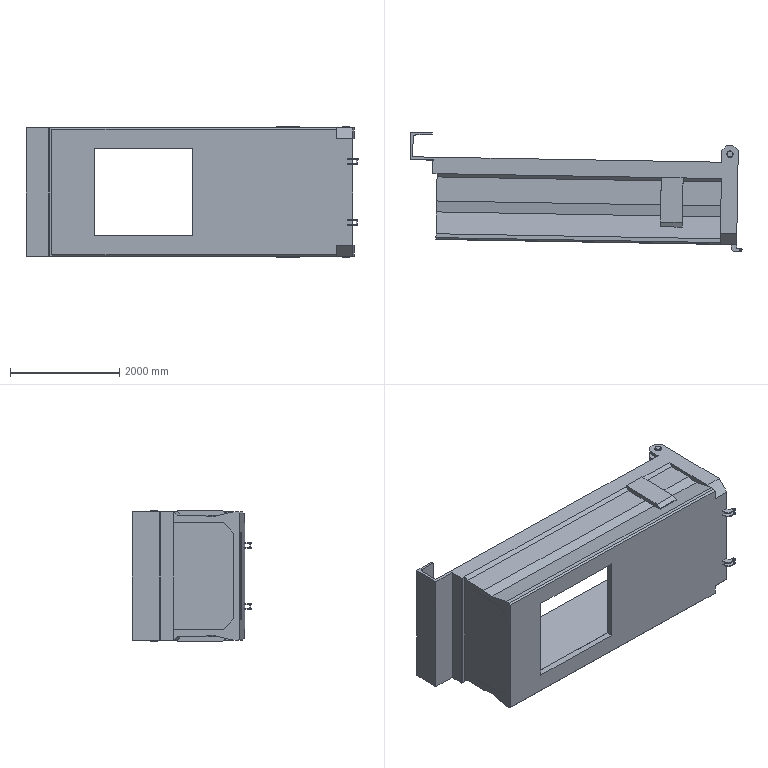Component | SolidWorks | CargoBox-1 | 3 solids | 192 faces | box 6072.17 x 2185.91 x 2410 mm | volume 3913118645 mm3 | plane 125 | cylinder 51 | cone 16 | commonest cylinder face diameters 40 x20 120 x8 30 x8 80 x6 20 x6 100 x3
build123d program:
from build123d import *

# Parameters (mm, degrees)
BOSS_EXTRUDE1_DEPTH      = 2600
SKETCH3_W                = 1950
SKETCH3_H                = 1400
BOSS_EXTRUDE2_DEPTH      = 8
SKETCH4_W                = 2350
SKETCH4_H                = 250
BOSS_EXTRUDE3_DEPTH      = 80
FILLET1_R                = 10
BOSS_EXTRUDE4_DEPTH      = 300
SKETCH6_W                = 400
SKETCH6_H                = 900
BOSS_EXTRUDE5_DEPTH      = 80
CHAMFER1_SIZE            = 50
CHAMFER1_SIZE2           = 86.603
CHAMFER2_SIZE            = 90
CHAMFER2_SIZE2           = 51.962
CUT_EXTRUDE1_DEPTH       = 390
CHAMFER3_SIZE            = 190
BOSS_EXTRUDE7_DEPTH      = 2350
FILLET2_R                = 50
CHAMFER4_SIZE            = 80
SKETCH11_W               = 80
SKETCH11_H               = 300
CUT_EXTRUDE2_DEPTH       = 390
SKETCH12_R               = 40
CUT_EXTRUDE3_DEPTH       = 4319.495
BOSS_EXTRUDE8_REACH      = 4214.054
SKETCH13_R               = 40
CHAMFER5_SIZE            = 30
BOSS_EXTRUDE9_DEPTH      = 20
SKETCH15_R               = 10
CUT_EXTRUDE4_DEPTH       = 4036.035
SKETCH16_R               = 60
BOSS_EXTRUDE10_DEPTH     = 30
BOSS_EXTRUDE12_START     = 200
SKETCH18_R               = 40
BOSS_EXTRUDE12_DEPTH     = 200
BOSS_EXTRUDE11_START     = 30
SKETCH17_R               = 60
BOSS_EXTRUDE11_DEPTH     = 30
CHAMFER6_SIZE            = 10
CHAMFER6_OF_MIRROR2_SIZE = 10
SKETCH19_R               = 15
BOSS_EXTRUDE13_DEPTH     = 10
SKETCH20_R               = 10
BOSS_EXTRUDE14_DEPTH     = 100
CHAMFER7_SIZE            = 2
CHAMFER7_OF_MIRROR9_SIZE = 2
LPATTERN1_COUNT          = 2
LPATTERN1_PITCH          = 1115
CUT_EXTRUDE5_DEPTH       = 3806.854
CUT_EXTRUDE5_DEPTH_BACK  = 3806.854
SKETCH23_W               = 1601
SKETCH23_H               = 1804


with BuildPart() as part:
    # Sketch1 → Boss-Extrude1 (new, symmetric)
    with BuildSketch(Plane.XY):
        Polygon((-975, 1400), (-975, 0), (975, 0), (975, 1400), (1175, 1400), (1175, 1100), (1115, 1040), (1115, 600), (1079.735, 400), (1175, 0), (1175, -100), (-1175, -100), (-1175, 0), (-1079.735, 400), (-1115, 600), (-1115, 1040), (-1175, 1100), (-1175, 1400), align=None)
    extrude(amount=BOSS_EXTRUDE1_DEPTH, both=True)

    # Sketch3 → Boss-Extrude2 (add)
    with BuildSketch(Plane(origin=(0, 0, -2600), x_dir=(-1, 0, 0), z_dir=(0, 0, -1))):
        with Locations((0, 700)):
            Rectangle(SKETCH3_W, SKETCH3_H)
    extrude(amount=-BOSS_EXTRUDE2_DEPTH)

    # Sketch5 → Boss-Extrude4 (add)
    with BuildSketch(Plane.XY.offset(2600)):
        Polygon((-1175, 1700), (-1175, 100), (-975, -100), (975, -100), (1175, 100), (1175, 1700), align=None)
    extrude(amount=BOSS_EXTRUDE4_DEPTH)

    # Sketch6 → Boss-Extrude5 (add)
    with BuildSketch(Plane.ZY.offset(1115)):
        with Locations((1700, 650)):
            Rectangle(SKETCH6_W, SKETCH6_H)
    boss_extrude5 = extrude(amount=BOSS_EXTRUDE5_DEPTH)

    # Mirror1: Boss-Extrude5 across plane
    add(boss_extrude5.mirror(Plane(origin=(0, 0, 0), x_dir=(0, 0, 1), z_dir=(1, 0, 0))))

    # Chamfer1
    chamfer1_edges = [part.edges().sort_by_distance(p)[0] for p in [
        (-1195, 200, 1700),
    ]]
    chamfer1_side = [part.faces().sort_by_distance(p)[0] for p in [
        (-1161.184, 200, 1700),
    ]]
    chamfer(chamfer1_edges, length=CHAMFER1_SIZE, length2=CHAMFER1_SIZE2, reference=chamfer1_side[0])

    # Chamfer2
    chamfer2_edges = [part.edges().sort_by_distance(p)[0] for p in [
        (1195, 200, 1700),
    ]]
    chamfer2_side = [part.faces().sort_by_distance(p)[0] for p in [
        (1195, 650, 1700),
    ]]
    chamfer(chamfer2_edges, length=CHAMFER2_SIZE, length2=CHAMFER2_SIZE2, reference=chamfer2_side[0])

    # Sketch7 → Cut-Extrude1 (cut)
    with BuildSketch(Plane.XY.offset(2900)):
        Polygon((-975, 1700), (-975, 182.843), (-792.157, 0), (792.157, 0), (975, 182.843), (975, 1700), align=None)
    extrude(amount=-CUT_EXTRUDE1_DEPTH, mode=Mode.SUBTRACT)

    # Chamfer3
    chamfer3_edges = [part.edges().sort_by_distance(p)[0] for p in [
        (975, 0, 4),
        (-975, 0, 4),
    ]]
    chamfer(chamfer3_edges, length=CHAMFER3_SIZE)



with BuildPart() as body_2:
    # Sketch4 → Boss-Extrude3 (new body)
    with BuildSketch(Plane(origin=(0, 0, -2600), x_dir=(-1, 0, 0), z_dir=(0, 0, -1))):
        with Locations((0, 1225)):
            Rectangle(SKETCH4_W, SKETCH4_H)
    extrude(amount=BOSS_EXTRUDE3_DEPTH)

    # Fillet1
    fillet1_edges = [body_2.edges().sort_by_distance(p)[0] for p in [
        (0, 1350, -2680),
        (0, 1100, -2680),
    ]]
    fillet(fillet1_edges, radius=FILLET1_R)


with BuildPart() as part_1:
    add(part.part)

    add(body_2.part)  # Boss-Extrude7 merges body 2
    # Sketch9 → Boss-Extrude7 (add)
    with BuildSketch(Plane(origin=(1175, 0, 0), x_dir=(0, 0, -1), z_dir=(1, 0, 0))):
        with BuildLine():
            Line((2600, 1350), (3100, 1350))
            Line((3100, 1350), (3100, 1850))
            Line((3100, 1850), (2700, 1850))
            Line((2700, 1850), (2700, 1820))
            Line((2700, 1820), (3002.617, 1804.141))
            ThreePointArc((3002.617, 1804.141), (3036.269, 1788.627), (3050, 1754.209))
            Line((3050, 1754.209), (3050, 1400))
            Line((3050, 1400), (2600, 1400))
            Line((2600, 1400), (2600, 1350))
        make_face()
    extrude(amount=-BOSS_EXTRUDE7_DEPTH)

    # Fillet2
    fillet2_edges = [part_1.edges().sort_by_distance(p)[0] for p in [
        (1175, 1835, -2700),
        (-1175, 1835, -2700),
    ]]
    fillet(fillet2_edges, radius=FILLET2_R)

    # Chamfer4
    chamfer4_edges = [part_1.edges().sort_by_distance(p)[0] for p in [
        (1075, 1700, 2600),
        (-1075, 1700, 2600),
        (1075, 1700, 2900),
        (-1075, 1700, 2900),
    ]]
    chamfer(chamfer4_edges, length=CHAMFER4_SIZE)

    # Sketch11 → Cut-Extrude2 (cut)
    with BuildSketch(Plane.XY.offset(2900)):
        with Locations((1075, 1550)):
            Rectangle(SKETCH11_W, SKETCH11_H)
        with Locations((-1075, 1550)):
            Rectangle(SKETCH11_W, SKETCH11_H)
    extrude(amount=-CUT_EXTRUDE2_DEPTH, mode=Mode.SUBTRACT)

    # Sketch12 → Cut-Extrude3 (cut, through all)
    with BuildSketch(Plane(origin=(1175, 0, 0), x_dir=(0, 0, -1), z_dir=(1, 0, 0))):
        with Locations((-2750, 1550)):
            Circle(SKETCH12_R)
    extrude(amount=-CUT_EXTRUDE3_DEPTH, mode=Mode.SUBTRACT)

    # Sketch13 → Boss-Extrude8 (add, up to next)
    with BuildSketch(Plane(origin=(-975, 0, 0), x_dir=(0, 0, -1), z_dir=(1, 0, 0)), mode=Mode.PRIVATE) as boss_extrude8_sk1:
        with Locations(Location((-2300, 1200, 0), (0, 0, 180))):
            Circle(SKETCH13_R)
    boss_extrude8_tool1 = extrude(boss_extrude8_sk1.sketch, amount=BOSS_EXTRUDE8_REACH, mode=Mode.PRIVATE) - part_1.part
    add(boss_extrude8_tool1.solids().sort_by_distance((-975, 1200, 2300))[0])

    # Chamfer5
    chamfer5_edges = [part_1.edges().sort_by_distance(p)[0] for p in [
        (-1175, -100, 0),
        (1175, -100, 0),
    ]]
    chamfer(chamfer5_edges, length=CHAMFER5_SIZE)

    # Sketch16 → Boss-Extrude10 (add)
    with BuildSketch(Plane.ZY.offset(1175)):
        with Locations(Location((2750, 1550, 0), (0, 0, 180))):
            Circle(SKETCH16_R)
    boss_extrude10 = extrude(amount=BOSS_EXTRUDE10_DEPTH)

    # Sketch18 → Boss-Extrude12 (add)
    with BuildSketch(Plane(origin=(-1175, 0, 0), x_dir=(0, 0, -1), z_dir=(1, 0, 0)).offset(BOSS_EXTRUDE12_START)):
        with Locations((-2750, 1550)):
            Circle(SKETCH18_R)
    boss_extrude12 = extrude(amount=-BOSS_EXTRUDE12_DEPTH)

    # Sketch17 → Boss-Extrude11 (add)
    with BuildSketch(Plane(origin=(-975, 0, 0), x_dir=(0, 0, -1), z_dir=(1, 0, 0)).offset(BOSS_EXTRUDE11_START)):
        with Locations((-2750, 1550)):
            Circle(SKETCH17_R)
    boss_extrude11 = extrude(amount=-BOSS_EXTRUDE11_DEPTH)

    # Chamfer6
    chamfer6_edges = [part_1.edges().sort_by_distance(p)[0] for p in [
        (-1205, 1550, 2810),
        (-945, 1550, 2810),
    ]]
    chamfer(chamfer6_edges, length=CHAMFER6_SIZE)

    # Mirror2: Boss-Extrude10, Boss-Extrude12, Boss-Extrude11 across plane
    add(boss_extrude10.mirror(Plane(origin=(0, 0, 0), x_dir=(0, 0, 1), z_dir=(1, 0, 0))))
    add(boss_extrude12.mirror(Plane(origin=(0, 0, 0), x_dir=(0, 0, 1), z_dir=(1, 0, 0))))
    add(boss_extrude11.mirror(Plane(origin=(0, 0, 0), x_dir=(0, 0, 1), z_dir=(1, 0, 0))))

    # Chamfer6 of Mirror2
    chamfer6_of_mirror2_edges = [part_1.edges().sort_by_distance(p)[0] for p in [
        (1205, 1550, 2810),
        (945, 1550, 2810),
    ]]
    chamfer(chamfer6_of_mirror2_edges, length=CHAMFER6_OF_MIRROR2_SIZE)

    # Sketch23 → Cut-Extrude5 (cut, two sides: drawn at the far end of the back side and taken through both)
    with BuildSketch(Plane(origin=(0, 0, 0), x_dir=(1, 0, 0), z_dir=(0, 1, 0)).offset(-CUT_EXTRUDE5_DEPTH_BACK)):
        with Locations((0, 926.743)):
            Rectangle(SKETCH23_W, SKETCH23_H)
    extrude(amount=CUT_EXTRUDE5_DEPTH + CUT_EXTRUDE5_DEPTH_BACK, mode=Mode.SUBTRACT)


with BuildPart() as body_2_2:
    # Sketch14 → Boss-Extrude9 (new body)
    with BuildSketch(Plane.ZY.offset(607.5)):
        with BuildLine():
            Line((2800, -100), (2900, -100))
            Line((2900, -100), (2900, -150))
            ThreePointArc((2900, -150), (2905.858, -164.142), (2920, -170))
            Line((2920, -170), (2980, -170))
            ThreePointArc((2980, -170), (2994.142, -175.858), (3000, -190))
            Line((3000, -190), (3000, -210))
            ThreePointArc((3000, -210), (2994.142, -224.142), (2980, -230))
            Line((2980, -230), (2858.284, -230))
            ThreePointArc((2858.284, -230), (2850.631, -228.478), (2844.142, -224.142))
            Line((2844.142, -224.142), (2805.858, -185.858))
            ThreePointArc((2805.858, -185.858), (2801.522, -179.369), (2800, -171.716))
            Line((2800, -171.716), (2800, -100))
        make_face()
    extrude(amount=-BOSS_EXTRUDE9_DEPTH)

    # Sketch15 → Cut-Extrude4 (cut, through all)
    with BuildSketch(Plane.ZY.offset(607.5)):
        with Locations((2975, -200)):
            Circle(SKETCH15_R)
    extrude(amount=-CUT_EXTRUDE4_DEPTH, mode=Mode.SUBTRACT)


with BuildPart() as body_3:
    # Body-Move_Copy1: copy of body 2 2
    add(body_2_2.part.moved(Location((80, 0, 0))))


with BuildPart() as body_2_2_1:
    add(body_2_2.part)

    # Sketch19 → Boss-Extrude13 (add)
    with BuildSketch(Plane.ZY.offset(607.5)):
        with Locations((2975, -200)):
            Circle(SKETCH19_R)
    boss_extrude13 = extrude(amount=BOSS_EXTRUDE13_DEPTH)

    add(body_3.part)  # Boss-Extrude14 merges body 3
    # Sketch20 → Boss-Extrude14 (add)
    with BuildSketch(Plane(origin=(-607.5, 0, 0), x_dir=(0, 0, -1), z_dir=(1, 0, 0))):
        with Locations(Location((-2975, -200, 0), (0, 0, 180))):
            Circle(SKETCH20_R)
    extrude(amount=BOSS_EXTRUDE14_DEPTH)

    # Chamfer7
    chamfer7_edges = [body_2_2_1.edges().sort_by_distance(p)[0] for p in [
        (-617.5, -200, 2960),
    ]]
    chamfer(chamfer7_edges, length=CHAMFER7_SIZE)

    # Mirror9: Boss-Extrude13 across plane
    add(boss_extrude13.mirror(Plane.ZY.offset(557.5)))

    # Chamfer7 of Mirror9
    chamfer7_of_mirror9_edges = [body_2_2_1.edges().sort_by_distance(p)[0] for p in [
        (-497.5, -200, 2960),
    ]]
    chamfer(chamfer7_of_mirror9_edges, length=CHAMFER7_OF_MIRROR9_SIZE)


with BuildPart() as lpattern1_1:
    # LPattern1: pattern copy
    add(body_2_2_1.part.moved(Location(Vector(1, 0, 0) * (1 * LPATTERN1_PITCH))))


solid = Compound([part_1.part, body_2_2_1.part, lpattern1_1.part])

# Placed as in the assembly
solid = solid.moved(Location((-1840.247, 1514.222, -62.386), (90, 88.999, -90)))